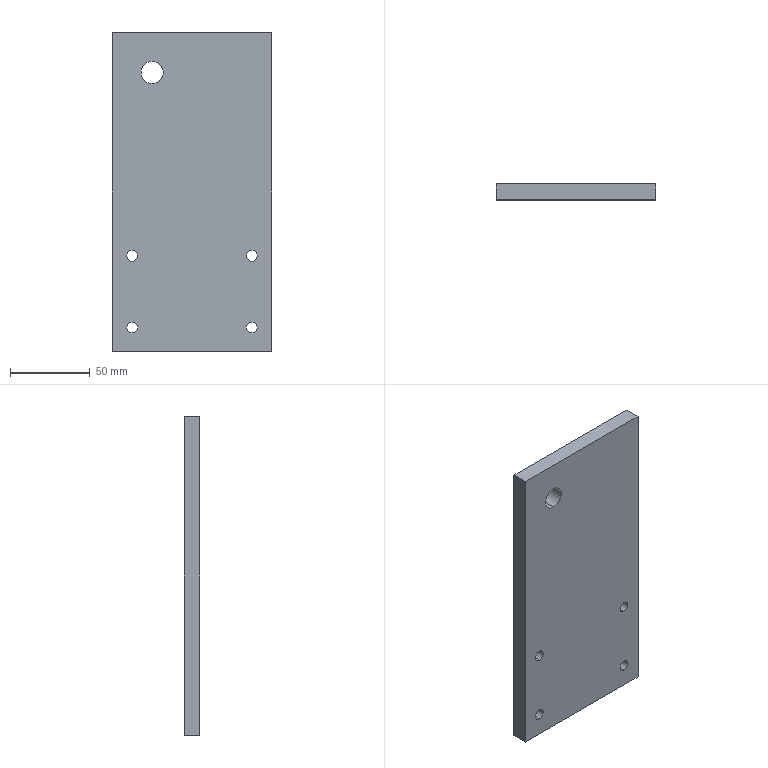Component | SolidWorks | FootPlate-1 | 1 solid | 16 faces | box 100 x 10 x 200 mm | volume 197008 mm3 | cylinder 10 | plane 6 | commonest cylinder face diameters 6.8 x8 14 x2
build123d program:
from build123d import *

# Parameters (mm, degrees)
SKETCH1_W           = 200
SKETCH1_H           = 100
BOSS_EXTRUDE1_DEPTH = 10
M16_TAPPED_HOLE1_D  = 14
M8_TAPPED_HOLE1_D   = 6.8


with BuildPart() as part:
    # Sketch1 → Boss-Extrude1 (new body)
    with BuildSketch(Plane.XY):
        Rectangle(SKETCH1_W, SKETCH1_H)
    extrude(amount=BOSS_EXTRUDE1_DEPTH)

    # M16 Tapped Hole1 (through all)
    with Locations(Plane.XY.offset(10)):
        with Locations((75, 25)):
            Hole(M16_TAPPED_HOLE1_D / 2)

    # M8 Tapped Hole1 (through all)
    with Locations(Plane.XY.offset(10)):
        with Locations((-85, 37.5), (-85, -37.5), (-40, -37.5), (-40, 37.5)):
            Hole(M8_TAPPED_HOLE1_D / 2)


solid = part.part

# Placed as in the assembly
solid = solid.moved(Location((-15.532, 1144.666, 2256.399), (90, 0, 90)))
STEP:
#1=COLOUR_RGB('',0.7922,0.8196,0.9333);
#2=FILL_AREA_STYLE_COLOUR('',#1);
#3=FILL_AREA_STYLE('',(#2));
#4=SURFACE_STYLE_FILL_AREA(#3);
#5=SURFACE_SIDE_STYLE('',(#4));
#6=SURFACE_STYLE_USAGE(.BOTH.,#5);
#7=PRESENTATION_STYLE_ASSIGNMENT((#6));
#8=CARTESIAN_POINT('',(-2.088,45.066,85.354));
#9=VERTEX_POINT('',#8);
#10=CARTESIAN_POINT('',(-2.088,45.066,85.622));
#11=VERTEX_POINT('',#10);
#12=CARTESIAN_POINT('',(-2.088,45.066,85.488));
#13=DIRECTION('',(0.,-1.,-0.));
#14=DIRECTION('',(0.,0.,1.));
#15=AXIS2_PLACEMENT_3D('',#12,#13,#14);
#16=CIRCLE('',#15,0.1339);
#17=EDGE_CURVE('',#9,#11,#16,.T.);
#18=ORIENTED_EDGE('',*,*,#17,.F.);
#19=CARTESIAN_POINT('',(-2.088,44.672,85.354));
#20=VERTEX_POINT('',#19);
#21=CARTESIAN_POINT('',(-2.088,44.672,85.354));
#22=DIRECTION('',(0.,-1.,-0.));
#23=VECTOR('',#22,39.37);
#24=LINE('',#21,#23);
#25=EDGE_CURVE('',#9,#20,#24,.T.);
#26=ORIENTED_EDGE('',*,*,#25,.T.);
#27=CARTESIAN_POINT('',(-2.088,44.672,85.622));
#28=VERTEX_POINT('',#27);
#29=CARTESIAN_POINT('',(-2.088,44.672,85.488));
#30=DIRECTION('',(0.,-1.,-0.));
#31=DIRECTION('',(0.,0.,1.));
#32=AXIS2_PLACEMENT_3D('',#29,#30,#31);
#33=CIRCLE('',#32,0.1339);
#34=EDGE_CURVE('',#20,#28,#33,.T.);
#35=ORIENTED_EDGE('',*,*,#34,.T.);
#36=CARTESIAN_POINT('',(-2.088,44.672,85.622));
#37=DIRECTION('',(0.,-1.,-0.));
#38=VECTOR('',#37,39.37);
#39=LINE('',#36,#38);
#40=EDGE_CURVE('',#11,#28,#39,.T.);
#41=ORIENTED_EDGE('',*,*,#40,.F.);
#42=EDGE_LOOP('',(#18,#26,#35,#41));
#43=FACE_OUTER_BOUND('',#42,.T.);
#44=CARTESIAN_POINT('',(-2.088,44.672,85.488));
#45=DIRECTION('',(0.,-1.,-0.));
#46=DIRECTION('',(0.,0.,1.));
#47=AXIS2_PLACEMENT_3D('',#44,#45,#46);
#48=CYLINDRICAL_SURFACE('',#47,0.1339);
#49=ADVANCED_FACE('',(#43),#48,.F.);
#50=CARTESIAN_POINT('',(0.8649,45.066,85.354));
#51=VERTEX_POINT('',#50);
#52=CARTESIAN_POINT('',(0.8649,45.066,85.622));
#53=VERTEX_POINT('',#52);
#54=CARTESIAN_POINT('',(0.8649,45.066,85.488));
#55=DIRECTION('',(0.,-1.,-0.));
#56=DIRECTION('',(0.,0.,1.));
#57=AXIS2_PLACEMENT_3D('',#54,#55,#56);
#58=CIRCLE('',#57,0.1339);
#59=EDGE_CURVE('',#51,#53,#58,.T.);
#60=ORIENTED_EDGE('',*,*,#59,.F.);
#61=CARTESIAN_POINT('',(0.8649,44.672,85.354));
#62=VERTEX_POINT('',#61);
#63=CARTESIAN_POINT('',(0.8649,44.672,85.354));
#64=DIRECTION('',(0.,-1.,-0.));
#65=VECTOR('',#64,39.37);
#66=LINE('',#63,#65);
#67=EDGE_CURVE('',#51,#62,#66,.T.);
#68=ORIENTED_EDGE('',*,*,#67,.T.);
#69=CARTESIAN_POINT('',(0.8649,44.672,85.622));
#70=VERTEX_POINT('',#69);
#71=CARTESIAN_POINT('',(0.8649,44.672,85.488));
#72=DIRECTION('',(0.,-1.,-0.));
#73=DIRECTION('',(0.,0.,1.));
#74=AXIS2_PLACEMENT_3D('',#71,#72,#73);
#75=CIRCLE('',#74,0.1339);
#76=EDGE_CURVE('',#62,#70,#75,.T.);
#77=ORIENTED_EDGE('',*,*,#76,.T.);
#78=CARTESIAN_POINT('',(0.8649,44.672,85.622));
#79=DIRECTION('',(0.,-1.,-0.));
#80=VECTOR('',#79,39.37);
#81=LINE('',#78,#80);
#82=EDGE_CURVE('',#53,#70,#81,.T.);
#83=ORIENTED_EDGE('',*,*,#82,.F.);
#84=EDGE_LOOP('',(#60,#68,#77,#83));
#85=FACE_OUTER_BOUND('',#84,.T.);
#86=CARTESIAN_POINT('',(0.8649,44.672,85.488));
#87=DIRECTION('',(0.,-1.,-0.));
#88=DIRECTION('',(0.,0.,1.));
#89=AXIS2_PLACEMENT_3D('',#86,#87,#88);
#90=CYLINDRICAL_SURFACE('',#89,0.1339);
#91=ADVANCED_FACE('',(#85),#90,.F.);
#92=CARTESIAN_POINT('',(0.8649,45.066,87.126));
#93=VERTEX_POINT('',#92);
#94=CARTESIAN_POINT('',(0.8649,45.066,87.394));
#95=VERTEX_POINT('',#94);
#96=CARTESIAN_POINT('',(0.8649,45.066,87.26));
#97=DIRECTION('',(0.,-1.,-0.));
#98=DIRECTION('',(0.,0.,1.));
#99=AXIS2_PLACEMENT_3D('',#96,#97,#98);
#100=CIRCLE('',#99,0.1339);
#101=EDGE_CURVE('',#93,#95,#100,.T.);
#102=ORIENTED_EDGE('',*,*,#101,.F.);
#103=CARTESIAN_POINT('',(0.8649,44.672,87.126));
#104=VERTEX_POINT('',#103);
#105=CARTESIAN_POINT('',(0.8649,44.672,87.126));
#106=DIRECTION('',(0.,-1.,-0.));
#107=VECTOR('',#106,39.37);
#108=LINE('',#105,#107);
#109=EDGE_CURVE('',#93,#104,#108,.T.);
#110=ORIENTED_EDGE('',*,*,#109,.T.);
#111=CARTESIAN_POINT('',(0.8649,44.672,87.394));
#112=VERTEX_POINT('',#111);
#113=CARTESIAN_POINT('',(0.8649,44.672,87.26));
#114=DIRECTION('',(0.,-1.,-0.));
#115=DIRECTION('',(0.,0.,1.));
#116=AXIS2_PLACEMENT_3D('',#113,#114,#115);
#117=CIRCLE('',#116,0.1339);
#118=EDGE_CURVE('',#104,#112,#117,.T.);
#119=ORIENTED_EDGE('',*,*,#118,.T.);
#120=CARTESIAN_POINT('',(0.8649,44.672,87.394));
#121=DIRECTION('',(0.,-1.,-0.));
#122=VECTOR('',#121,39.37);
#123=LINE('',#120,#122);
#124=EDGE_CURVE('',#95,#112,#123,.T.);
#125=ORIENTED_EDGE('',*,*,#124,.F.);
#126=EDGE_LOOP('',(#102,#110,#119,#125));
#127=FACE_OUTER_BOUND('',#126,.T.);
#128=CARTESIAN_POINT('',(0.8649,44.672,87.26));
#129=DIRECTION('',(0.,-1.,-0.));
#130=DIRECTION('',(0.,0.,1.));
#131=AXIS2_PLACEMENT_3D('',#128,#129,#130);
#132=CYLINDRICAL_SURFACE('',#131,0.1339);
#133=ADVANCED_FACE('',(#127),#132,.F.);
#134=CARTESIAN_POINT('',(-2.088,45.066,87.126));
#135=VERTEX_POINT('',#134);
#136=CARTESIAN_POINT('',(-2.088,45.066,87.394));
#137=VERTEX_POINT('',#136);
#138=CARTESIAN_POINT('',(-2.088,45.066,87.26));
#139=DIRECTION('',(0.,-1.,-0.));
#140=DIRECTION('',(0.,0.,1.));
#141=AXIS2_PLACEMENT_3D('',#138,#139,#140);
#142=CIRCLE('',#141,0.1339);
#143=EDGE_CURVE('',#135,#137,#142,.T.);
#144=ORIENTED_EDGE('',*,*,#143,.F.);
#145=CARTESIAN_POINT('',(-2.088,44.672,87.126));
#146=VERTEX_POINT('',#145);
#147=CARTESIAN_POINT('',(-2.088,44.672,87.126));
#148=DIRECTION('',(0.,-1.,-0.));
#149=VECTOR('',#148,39.37);
#150=LINE('',#147,#149);
#151=EDGE_CURVE('',#135,#146,#150,.T.);
#152=ORIENTED_EDGE('',*,*,#151,.T.);
#153=CARTESIAN_POINT('',(-2.088,44.672,87.394));
#154=VERTEX_POINT('',#153);
#155=CARTESIAN_POINT('',(-2.088,44.672,87.26));
#156=DIRECTION('',(0.,-1.,-0.));
#157=DIRECTION('',(0.,0.,1.));
#158=AXIS2_PLACEMENT_3D('',#155,#156,#157);
#159=CIRCLE('',#158,0.1339);
#160=EDGE_CURVE('',#146,#154,#159,.T.);
#161=ORIENTED_EDGE('',*,*,#160,.T.);
#162=CARTESIAN_POINT('',(-2.088,44.672,87.394));
#163=DIRECTION('',(0.,-1.,-0.));
#164=VECTOR('',#163,39.37);
#165=LINE('',#162,#164);
#166=EDGE_CURVE('',#137,#154,#165,.T.);
#167=ORIENTED_EDGE('',*,*,#166,.F.);
#168=EDGE_LOOP('',(#144,#152,#161,#167));
#169=FACE_OUTER_BOUND('',#168,.T.);
#170=CARTESIAN_POINT('',(-2.088,44.672,87.26));
#171=DIRECTION('',(0.,-1.,-0.));
#172=DIRECTION('',(0.,0.,1.));
#173=AXIS2_PLACEMENT_3D('',#170,#171,#172);
#174=CYLINDRICAL_SURFACE('',#173,0.1339);
#175=ADVANCED_FACE('',(#169),#174,.F.);
#176=CARTESIAN_POINT('',(-1.596,45.066,91.512));
#177=VERTEX_POINT('',#176);
#178=CARTESIAN_POINT('',(-1.596,45.066,92.063));
#179=VERTEX_POINT('',#178);
#180=CARTESIAN_POINT('',(-1.596,45.066,91.787));
#181=DIRECTION('',(0.,-1.,-0.));
#182=DIRECTION('',(0.,0.,1.));
#183=AXIS2_PLACEMENT_3D('',#180,#181,#182);
#184=CIRCLE('',#183,0.2756);
#185=EDGE_CURVE('',#177,#179,#184,.T.);
#186=ORIENTED_EDGE('',*,*,#185,.F.);
#187=CARTESIAN_POINT('',(-1.596,44.672,91.512));
#188=VERTEX_POINT('',#187);
#189=CARTESIAN_POINT('',(-1.596,44.672,91.512));
#190=DIRECTION('',(0.,-1.,-0.));
#191=VECTOR('',#190,39.37);
#192=LINE('',#189,#191);
#193=EDGE_CURVE('',#177,#188,#192,.T.);
#194=ORIENTED_EDGE('',*,*,#193,.T.);
#195=CARTESIAN_POINT('',(-1.596,44.672,92.063));
#196=VERTEX_POINT('',#195);
#197=CARTESIAN_POINT('',(-1.596,44.672,91.787));
#198=DIRECTION('',(0.,-1.,-0.));
#199=DIRECTION('',(0.,0.,1.));
#200=AXIS2_PLACEMENT_3D('',#197,#198,#199);
#201=CIRCLE('',#200,0.2756);
#202=EDGE_CURVE('',#188,#196,#201,.T.);
#203=ORIENTED_EDGE('',*,*,#202,.T.);
#204=CARTESIAN_POINT('',(-1.596,44.672,92.063));
#205=DIRECTION('',(0.,-1.,-0.));
#206=VECTOR('',#205,39.37);
#207=LINE('',#204,#206);
#208=EDGE_CURVE('',#179,#196,#207,.T.);
#209=ORIENTED_EDGE('',*,*,#208,.F.);
#210=EDGE_LOOP('',(#186,#194,#203,#209));
#211=FACE_OUTER_BOUND('',#210,.T.);
#212=CARTESIAN_POINT('',(-1.596,44.672,91.787));
#213=DIRECTION('',(0.,-1.,-0.));
#214=DIRECTION('',(0.,0.,1.));
#215=AXIS2_PLACEMENT_3D('',#212,#213,#214);
#216=CYLINDRICAL_SURFACE('',#215,0.2756);
#217=ADVANCED_FACE('',(#211),#216,.F.);
#218=CARTESIAN_POINT('',(1.357,45.066,92.772));
#219=VERTEX_POINT('',#218);
#220=CARTESIAN_POINT('',(-2.58,45.066,92.772));
#221=VERTEX_POINT('',#220);
#222=CARTESIAN_POINT('',(-2.58,45.066,92.772));
#223=DIRECTION('',(-1.,-0.,-0.));
#224=VECTOR('',#223,39.37);
#225=LINE('',#222,#224);
#226=EDGE_CURVE('',#219,#221,#225,.T.);
#227=ORIENTED_EDGE('',*,*,#226,.T.);
#228=CARTESIAN_POINT('',(-2.58,44.672,92.772));
#229=VERTEX_POINT('',#228);
#230=CARTESIAN_POINT('',(-2.58,44.672,92.772));
#231=DIRECTION('',(-0.,1.,0.));
#232=VECTOR('',#231,39.37);
#233=LINE('',#230,#232);
#234=EDGE_CURVE('',#229,#221,#233,.T.);
#235=ORIENTED_EDGE('',*,*,#234,.F.);
#236=CARTESIAN_POINT('',(1.357,44.672,92.772));
#237=VERTEX_POINT('',#236);
#238=CARTESIAN_POINT('',(-2.58,44.672,92.772));
#239=DIRECTION('',(-1.,-0.,-0.));
#240=VECTOR('',#239,39.37);
#241=LINE('',#238,#240);
#242=EDGE_CURVE('',#237,#229,#241,.T.);
#243=ORIENTED_EDGE('',*,*,#242,.F.);
#244=CARTESIAN_POINT('',(1.357,44.672,92.772));
#245=DIRECTION('',(-0.,1.,0.));
#246=VECTOR('',#245,39.37);
#247=LINE('',#244,#246);
#248=EDGE_CURVE('',#237,#219,#247,.T.);
#249=ORIENTED_EDGE('',*,*,#248,.T.);
#250=EDGE_LOOP('',(#227,#235,#243,#249));
#251=FACE_OUTER_BOUND('',#250,.T.);
#252=CARTESIAN_POINT('',(-2.58,44.672,92.772));
#253=DIRECTION('',(0.,0.,-1.));
#254=DIRECTION('',(0.,-1.,-0.));
#255=AXIS2_PLACEMENT_3D('',#252,#253,#254);
#256=PLANE('',#255);
#257=ADVANCED_FACE('',(#251),#256,.F.);
#258=CARTESIAN_POINT('',(-2.58,45.066,84.898));
#259=VERTEX_POINT('',#258);
#260=CARTESIAN_POINT('',(-2.58,45.066,84.898));
#261=DIRECTION('',(0.,-0.,-1.));
#262=VECTOR('',#261,39.37);
#263=LINE('',#260,#262);
#264=EDGE_CURVE('',#221,#259,#263,.T.);
#265=ORIENTED_EDGE('',*,*,#264,.T.);
#266=CARTESIAN_POINT('',(-2.58,44.672,84.898));
#267=VERTEX_POINT('',#266);
#268=CARTESIAN_POINT('',(-2.58,44.672,84.898));
#269=DIRECTION('',(-0.,1.,0.));
#270=VECTOR('',#269,39.37);
#271=LINE('',#268,#270);
#272=EDGE_CURVE('',#267,#259,#271,.T.);
#273=ORIENTED_EDGE('',*,*,#272,.F.);
#274=CARTESIAN_POINT('',(-2.58,44.672,84.898));
#275=DIRECTION('',(0.,-0.,-1.));
#276=VECTOR('',#275,39.37);
#277=LINE('',#274,#276);
#278=EDGE_CURVE('',#229,#267,#277,.T.);
#279=ORIENTED_EDGE('',*,*,#278,.F.);
#280=ORIENTED_EDGE('',*,*,#234,.T.);
#281=EDGE_LOOP('',(#265,#273,#279,#280));
#282=FACE_OUTER_BOUND('',#281,.T.);
#283=CARTESIAN_POINT('',(-2.58,44.672,84.898));
#284=DIRECTION('',(1.,0.,0.));
#285=DIRECTION('',(-0.,1.,0.));
#286=AXIS2_PLACEMENT_3D('',#283,#284,#285);
#287=PLANE('',#286);
#288=ADVANCED_FACE('',(#282),#287,.F.);
#289=CARTESIAN_POINT('',(1.357,45.066,84.898));
#290=VERTEX_POINT('',#289);
#291=CARTESIAN_POINT('',(-2.58,45.066,84.898));
#292=DIRECTION('',(1.,0.,0.));
#293=VECTOR('',#292,39.37);
#294=LINE('',#291,#293);
#295=EDGE_CURVE('',#259,#290,#294,.T.);
#296=ORIENTED_EDGE('',*,*,#295,.T.);
#297=CARTESIAN_POINT('',(1.357,44.672,84.898));
#298=VERTEX_POINT('',#297);
#299=CARTESIAN_POINT('',(1.357,44.672,84.898));
#300=DIRECTION('',(-0.,1.,0.));
#301=VECTOR('',#300,39.37);
#302=LINE('',#299,#301);
#303=EDGE_CURVE('',#298,#290,#302,.T.);
#304=ORIENTED_EDGE('',*,*,#303,.F.);
#305=CARTESIAN_POINT('',(-2.58,44.672,84.898));
#306=DIRECTION('',(1.,0.,0.));
#307=VECTOR('',#306,39.37);
#308=LINE('',#305,#307);
#309=EDGE_CURVE('',#267,#298,#308,.T.);
#310=ORIENTED_EDGE('',*,*,#309,.F.);
#311=ORIENTED_EDGE('',*,*,#272,.T.);
#312=EDGE_LOOP('',(#296,#304,#310,#311));
#313=FACE_OUTER_BOUND('',#312,.T.);
#314=CARTESIAN_POINT('',(-2.58,44.672,84.898));
#315=DIRECTION('',(-0.,0.,1.));
#316=DIRECTION('',(-1.,-0.,-0.));
#317=AXIS2_PLACEMENT_3D('',#314,#315,#316);
#318=PLANE('',#317);
#319=ADVANCED_FACE('',(#313),#318,.F.);
#320=CARTESIAN_POINT('',(1.357,45.066,84.898));
#321=DIRECTION('',(-0.,0.,1.));
#322=VECTOR('',#321,39.37);
#323=LINE('',#320,#322);
#324=EDGE_CURVE('',#290,#219,#323,.T.);
#325=ORIENTED_EDGE('',*,*,#324,.T.);
#326=ORIENTED_EDGE('',*,*,#248,.F.);
#327=CARTESIAN_POINT('',(1.357,44.672,84.898));
#328=DIRECTION('',(-0.,0.,1.));
#329=VECTOR('',#328,39.37);
#330=LINE('',#327,#329);
#331=EDGE_CURVE('',#298,#237,#330,.T.);
#332=ORIENTED_EDGE('',*,*,#331,.F.);
#333=ORIENTED_EDGE('',*,*,#303,.T.);
#334=EDGE_LOOP('',(#325,#326,#332,#333));
#335=FACE_OUTER_BOUND('',#334,.T.);
#336=CARTESIAN_POINT('',(1.357,44.672,84.898));
#337=DIRECTION('',(-1.,-0.,-0.));
#338=DIRECTION('',(0.,-1.,-0.));
#339=AXIS2_PLACEMENT_3D('',#336,#337,#338);
#340=PLANE('',#339);
#341=ADVANCED_FACE('',(#335),#340,.F.);
#342=CARTESIAN_POINT('',(-2.088,44.672,85.488));
#343=DIRECTION('',(0.,-1.,-0.));
#344=DIRECTION('',(0.,0.,1.));
#345=AXIS2_PLACEMENT_3D('',#342,#343,#344);
#346=CIRCLE('',#345,0.1339);
#347=EDGE_CURVE('',#28,#20,#346,.T.);
#348=ORIENTED_EDGE('',*,*,#347,.F.);
#349=ORIENTED_EDGE('',*,*,#34,.F.);
#350=EDGE_LOOP('',(#348,#349));
#351=FACE_BOUND('',#350,.T.);
#352=CARTESIAN_POINT('',(0.8649,44.672,85.488));
#353=DIRECTION('',(0.,-1.,-0.));
#354=DIRECTION('',(0.,0.,1.));
#355=AXIS2_PLACEMENT_3D('',#352,#353,#354);
#356=CIRCLE('',#355,0.1339);
#357=EDGE_CURVE('',#70,#62,#356,.T.);
#358=ORIENTED_EDGE('',*,*,#357,.F.);
#359=ORIENTED_EDGE('',*,*,#76,.F.);
#360=EDGE_LOOP('',(#358,#359));
#361=FACE_BOUND('',#360,.T.);
#362=CARTESIAN_POINT('',(0.8649,44.672,87.26));
#363=DIRECTION('',(0.,-1.,-0.));
#364=DIRECTION('',(0.,0.,1.));
#365=AXIS2_PLACEMENT_3D('',#362,#363,#364);
#366=CIRCLE('',#365,0.1339);
#367=EDGE_CURVE('',#112,#104,#366,.T.);
#368=ORIENTED_EDGE('',*,*,#367,.F.);
#369=ORIENTED_EDGE('',*,*,#118,.F.);
#370=EDGE_LOOP('',(#368,#369));
#371=FACE_BOUND('',#370,.T.);
#372=CARTESIAN_POINT('',(-2.088,44.672,87.26));
#373=DIRECTION('',(0.,-1.,-0.));
#374=DIRECTION('',(0.,0.,1.));
#375=AXIS2_PLACEMENT_3D('',#372,#373,#374);
#376=CIRCLE('',#375,0.1339);
#377=EDGE_CURVE('',#154,#146,#376,.T.);
#378=ORIENTED_EDGE('',*,*,#377,.F.);
#379=ORIENTED_EDGE('',*,*,#160,.F.);
#380=EDGE_LOOP('',(#378,#379));
#381=FACE_BOUND('',#380,.T.);
#382=CARTESIAN_POINT('',(-1.596,44.672,91.787));
#383=DIRECTION('',(0.,-1.,-0.));
#384=DIRECTION('',(0.,0.,1.));
#385=AXIS2_PLACEMENT_3D('',#382,#383,#384);
#386=CIRCLE('',#385,0.2756);
#387=EDGE_CURVE('',#196,#188,#386,.T.);
#388=ORIENTED_EDGE('',*,*,#387,.F.);
#389=ORIENTED_EDGE('',*,*,#202,.F.);
#390=EDGE_LOOP('',(#388,#389));
#391=FACE_BOUND('',#390,.T.);
#392=ORIENTED_EDGE('',*,*,#242,.T.);
#393=ORIENTED_EDGE('',*,*,#278,.T.);
#394=ORIENTED_EDGE('',*,*,#309,.T.);
#395=ORIENTED_EDGE('',*,*,#331,.T.);
#396=EDGE_LOOP('',(#392,#393,#394,#395));
#397=FACE_OUTER_BOUND('',#396,.T.);
#398=CARTESIAN_POINT('',(-0.6115,44.672,88.835));
#399=DIRECTION('',(0.,-1.,0.));
#400=DIRECTION('',(-0.,0.,1.));
#401=AXIS2_PLACEMENT_3D('',#398,#399,#400);
#402=PLANE('',#401);
#403=ADVANCED_FACE('',(#351,#361,#371,#381,#391,#397),#402,.T.);
#404=CARTESIAN_POINT('',(-2.088,45.066,85.488));
#405=DIRECTION('',(0.,-1.,-0.));
#406=DIRECTION('',(0.,0.,1.));
#407=AXIS2_PLACEMENT_3D('',#404,#405,#406);
#408=CIRCLE('',#407,0.1339);
#409=EDGE_CURVE('',#11,#9,#408,.T.);
#410=ORIENTED_EDGE('',*,*,#409,.T.);
#411=ORIENTED_EDGE('',*,*,#17,.T.);
#412=EDGE_LOOP('',(#410,#411));
#413=FACE_BOUND('',#412,.T.);
#414=CARTESIAN_POINT('',(0.8649,45.066,85.488));
#415=DIRECTION('',(0.,-1.,-0.));
#416=DIRECTION('',(0.,0.,1.));
#417=AXIS2_PLACEMENT_3D('',#414,#415,#416);
#418=CIRCLE('',#417,0.1339);
#419=EDGE_CURVE('',#53,#51,#418,.T.);
#420=ORIENTED_EDGE('',*,*,#419,.T.);
#421=ORIENTED_EDGE('',*,*,#59,.T.);
#422=EDGE_LOOP('',(#420,#421));
#423=FACE_BOUND('',#422,.T.);
#424=CARTESIAN_POINT('',(0.8649,45.066,87.26));
#425=DIRECTION('',(0.,-1.,-0.));
#426=DIRECTION('',(0.,0.,1.));
#427=AXIS2_PLACEMENT_3D('',#424,#425,#426);
#428=CIRCLE('',#427,0.1339);
#429=EDGE_CURVE('',#95,#93,#428,.T.);
#430=ORIENTED_EDGE('',*,*,#429,.T.);
#431=ORIENTED_EDGE('',*,*,#101,.T.);
#432=EDGE_LOOP('',(#430,#431));
#433=FACE_BOUND('',#432,.T.);
#434=CARTESIAN_POINT('',(-2.088,45.066,87.26));
#435=DIRECTION('',(0.,-1.,-0.));
#436=DIRECTION('',(0.,0.,1.));
#437=AXIS2_PLACEMENT_3D('',#434,#435,#436);
#438=CIRCLE('',#437,0.1339);
#439=EDGE_CURVE('',#137,#135,#438,.T.);
#440=ORIENTED_EDGE('',*,*,#439,.T.);
#441=ORIENTED_EDGE('',*,*,#143,.T.);
#442=EDGE_LOOP('',(#440,#441));
#443=FACE_BOUND('',#442,.T.);
#444=CARTESIAN_POINT('',(-1.596,45.066,91.787));
#445=DIRECTION('',(0.,-1.,-0.));
#446=DIRECTION('',(0.,0.,1.));
#447=AXIS2_PLACEMENT_3D('',#444,#445,#446);
#448=CIRCLE('',#447,0.2756);
#449=EDGE_CURVE('',#179,#177,#448,.T.);
#450=ORIENTED_EDGE('',*,*,#449,.T.);
#451=ORIENTED_EDGE('',*,*,#185,.T.);
#452=EDGE_LOOP('',(#450,#451));
#453=FACE_BOUND('',#452,.T.);
#454=ORIENTED_EDGE('',*,*,#226,.F.);
#455=ORIENTED_EDGE('',*,*,#324,.F.);
#456=ORIENTED_EDGE('',*,*,#295,.F.);
#457=ORIENTED_EDGE('',*,*,#264,.F.);
#458=EDGE_LOOP('',(#454,#455,#456,#457));
#459=FACE_OUTER_BOUND('',#458,.T.);
#460=CARTESIAN_POINT('',(-0.6115,45.066,88.835));
#461=DIRECTION('',(0.,-1.,0.));
#462=DIRECTION('',(-0.,0.,1.));
#463=AXIS2_PLACEMENT_3D('',#460,#461,#462);
#464=PLANE('',#463);
#465=ADVANCED_FACE('',(#413,#423,#433,#443,#453,#459),#464,.F.);
#466=ORIENTED_EDGE('',*,*,#193,.F.);
#467=ORIENTED_EDGE('',*,*,#449,.F.);
#468=ORIENTED_EDGE('',*,*,#208,.T.);
#469=ORIENTED_EDGE('',*,*,#387,.T.);
#470=EDGE_LOOP('',(#466,#467,#468,#469));
#471=FACE_OUTER_BOUND('',#470,.T.);
#472=CARTESIAN_POINT('',(-1.596,44.672,91.787));
#473=DIRECTION('',(0.,-1.,-0.));
#474=DIRECTION('',(0.,0.,1.));
#475=AXIS2_PLACEMENT_3D('',#472,#473,#474);
#476=CYLINDRICAL_SURFACE('',#475,0.2756);
#477=ADVANCED_FACE('',(#471),#476,.F.);
#478=ORIENTED_EDGE('',*,*,#151,.F.);
#479=ORIENTED_EDGE('',*,*,#439,.F.);
#480=ORIENTED_EDGE('',*,*,#166,.T.);
#481=ORIENTED_EDGE('',*,*,#377,.T.);
#482=EDGE_LOOP('',(#478,#479,#480,#481));
#483=FACE_OUTER_BOUND('',#482,.T.);
#484=CARTESIAN_POINT('',(-2.088,44.672,87.26));
#485=DIRECTION('',(0.,-1.,-0.));
#486=DIRECTION('',(0.,0.,1.));
#487=AXIS2_PLACEMENT_3D('',#484,#485,#486);
#488=CYLINDRICAL_SURFACE('',#487,0.1339);
#489=ADVANCED_FACE('',(#483),#488,.F.);
#490=ORIENTED_EDGE('',*,*,#109,.F.);
#491=ORIENTED_EDGE('',*,*,#429,.F.);
#492=ORIENTED_EDGE('',*,*,#124,.T.);
#493=ORIENTED_EDGE('',*,*,#367,.T.);
#494=EDGE_LOOP('',(#490,#491,#492,#493));
#495=FACE_OUTER_BOUND('',#494,.T.);
#496=CARTESIAN_POINT('',(0.8649,44.672,87.26));
#497=DIRECTION('',(0.,-1.,-0.));
#498=DIRECTION('',(0.,0.,1.));
#499=AXIS2_PLACEMENT_3D('',#496,#497,#498);
#500=CYLINDRICAL_SURFACE('',#499,0.1339);
#501=ADVANCED_FACE('',(#495),#500,.F.);
#502=ORIENTED_EDGE('',*,*,#67,.F.);
#503=ORIENTED_EDGE('',*,*,#419,.F.);
#504=ORIENTED_EDGE('',*,*,#82,.T.);
#505=ORIENTED_EDGE('',*,*,#357,.T.);
#506=EDGE_LOOP('',(#502,#503,#504,#505));
#507=FACE_OUTER_BOUND('',#506,.T.);
#508=CARTESIAN_POINT('',(0.8649,44.672,85.488));
#509=DIRECTION('',(0.,-1.,-0.));
#510=DIRECTION('',(0.,0.,1.));
#511=AXIS2_PLACEMENT_3D('',#508,#509,#510);
#512=CYLINDRICAL_SURFACE('',#511,0.1339);
#513=ADVANCED_FACE('',(#507),#512,.F.);
#514=ORIENTED_EDGE('',*,*,#25,.F.);
#515=ORIENTED_EDGE('',*,*,#409,.F.);
#516=ORIENTED_EDGE('',*,*,#40,.T.);
#517=ORIENTED_EDGE('',*,*,#347,.T.);
#518=EDGE_LOOP('',(#514,#515,#516,#517));
#519=FACE_OUTER_BOUND('',#518,.T.);
#520=CARTESIAN_POINT('',(-2.088,44.672,85.488));
#521=DIRECTION('',(0.,-1.,-0.));
#522=DIRECTION('',(0.,0.,1.));
#523=AXIS2_PLACEMENT_3D('',#520,#521,#522);
#524=CYLINDRICAL_SURFACE('',#523,0.1339);
#525=ADVANCED_FACE('',(#519),#524,.F.);
#526=CLOSED_SHELL('',(#49,#91,#133,#175,#217,#257,#288,#319,#341,#403,#465,#477,#489,#501,#513,#525));
#527=MANIFOLD_SOLID_BREP('',#526);
#528=STYLED_ITEM('',(#7),#527);
#529=PRESENTATION_LAYER_ASSIGNMENT('','',(#528));
#530=(LENGTH_UNIT()NAMED_UNIT(*)SI_UNIT($,.METRE.));
#531=LENGTH_MEASURE_WITH_UNIT(LENGTH_MEASURE(0.0254),#530);
#532=DIMENSIONAL_EXPONENTS(1.,0.,0.,0.,0.,0.,0.);
#533=(CONVERSION_BASED_UNIT('',#531)LENGTH_UNIT()NAMED_UNIT(#532));
#534=UNCERTAINTY_MEASURE_WITH_UNIT(LENGTH_MEASURE(0.00001),#533,'','');
#535=(NAMED_UNIT(*)PLANE_ANGLE_UNIT()SI_UNIT($,.RADIAN.));
#536=(NAMED_UNIT(*)SI_UNIT($,.STERADIAN.)SOLID_ANGLE_UNIT());
#537=(GEOMETRIC_REPRESENTATION_CONTEXT(3)GLOBAL_UNCERTAINTY_ASSIGNED_CONTEXT((#534))GLOBAL_UNIT_ASSIGNED_CONTEXT((#533,#535,#536))REPRESENTATION_CONTEXT('',''));
#538=MECHANICAL_DESIGN_GEOMETRIC_PRESENTATION_REPRESENTATION('',(#528),#537);
#539=CARTESIAN_POINT('',(0.,0.,0.));
#540=DIRECTION('',(0.,0.,1.));
#541=DIRECTION('',(1.,0.,0.));
#542=AXIS2_PLACEMENT_3D('',#539,#540,#541);
#543=(LENGTH_UNIT()NAMED_UNIT(*)SI_UNIT($,.METRE.));
#544=LENGTH_MEASURE_WITH_UNIT(LENGTH_MEASURE(0.0254),#543);
#545=DIMENSIONAL_EXPONENTS(1.,0.,0.,0.,0.,0.,0.);
#546=(CONVERSION_BASED_UNIT('',#544)LENGTH_UNIT()NAMED_UNIT(#545));
#547=UNCERTAINTY_MEASURE_WITH_UNIT(LENGTH_MEASURE(0.00001),#546,'','');
#548=(NAMED_UNIT(*)PLANE_ANGLE_UNIT()SI_UNIT($,.RADIAN.));
#549=(NAMED_UNIT(*)SI_UNIT($,.STERADIAN.)SOLID_ANGLE_UNIT());
#550=(GEOMETRIC_REPRESENTATION_CONTEXT(3)GLOBAL_UNCERTAINTY_ASSIGNED_CONTEXT((#547))GLOBAL_UNIT_ASSIGNED_CONTEXT((#546,#548,#549))REPRESENTATION_CONTEXT('',''));
#551=ADVANCED_BREP_SHAPE_REPRESENTATION('',(#527,#542),#550);